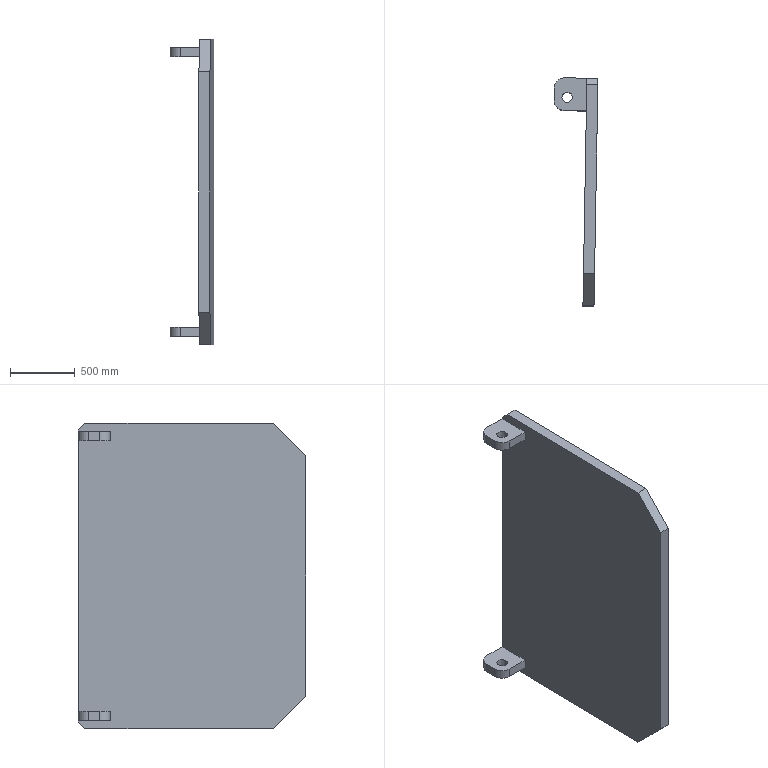Component | SolidWorks | BoxDoor-1 | 1 solid | 26 faces | box 337.93 x 1754.2 x 2350 mm | volume 351699217 mm3 | plane 18 | cylinder 8 | commonest cylinder face diameters 80 x4 160 x4
build123d program:
from build123d import *

# Parameters (mm, degrees)
BOSS_EXTRUDE1_DEPTH = 85
SKETCH2_W           = 70
SKETCH2_H           = 250
BOSS_EXTRUDE2_DEPTH = 250
CHAMFER1_SIZE       = 50
FILLET1_R           = 80
SKETCH3_R           = 40
CUT_EXTRUDE1_DEPTH  = 2460.543


with BuildPart() as part:
    # Sketch1 → Boss-Extrude1 (new body)
    with BuildSketch(Plane.XY):
        Polygon((-1175, -625), (-925, -875), (925, -875), (1175, -625), (1175, 875), (-1175, 875), align=None)
    extrude(amount=BOSS_EXTRUDE1_DEPTH)

    # Sketch2 → Boss-Extrude2 (add)
    with BuildSketch(Plane(origin=(0, 0, 0), x_dir=(-1, 0, 0), z_dir=(0, 0, -1))):
        with Locations((-1075, 750)):
            Rectangle(SKETCH2_W, SKETCH2_H)
        with Locations((1075, 750)):
            Rectangle(SKETCH2_W, SKETCH2_H)
    extrude(amount=BOSS_EXTRUDE2_DEPTH)

    # Chamfer1
    chamfer1_edges = [part.edges().sort_by_distance(p)[0] for p in [
        (-1175, 875, 42.5),
        (1175, 875, 42.5),
    ]]
    chamfer(chamfer1_edges, length=CHAMFER1_SIZE)

    # Fillet1
    fillet1_edges = [part.edges().sort_by_distance(p)[0] for p in [
        (1075, 625, -250),
        (1075, 875, -250),
        (-1075, 875, -250),
        (-1075, 625, -250),
    ]]
    fillet(fillet1_edges, radius=FILLET1_R)

    # Sketch3 → Cut-Extrude1 (cut, through all)
    with BuildSketch(Plane(origin=(1110, 0, 0), x_dir=(0, 0, -1), z_dir=(1, 0, 0))):
        with Locations(Location((150, 725, 0), (0, 0, 90))):
            Circle(SKETCH3_R)
    extrude(amount=-CUT_EXTRUDE1_DEPTH, mode=Mode.SUBTRACT)


solid = part.part

# Placed as in the assembly
solid = solid.moved(Location((1073.724, 2288.43, -62.386), (90, 88.999, -90)))
STEP:
#1=COLOUR_RGB('',0.7922,0.8196,0.9333);
#2=FILL_AREA_STYLE_COLOUR('',#1);
#3=FILL_AREA_STYLE('',(#2));
#4=SURFACE_STYLE_FILL_AREA(#3);
#5=SURFACE_SIDE_STYLE('',(#4));
#6=SURFACE_STYLE_USAGE(.BOTH.,#5);
#7=PRESENTATION_STYLE_ASSIGNMENT((#6));
#8=CARTESIAN_POINT('',(38.441,118.71,-43.401));
#9=VERTEX_POINT('',#8);
#10=CARTESIAN_POINT('',(35.292,118.765,-43.401));
#11=VERTEX_POINT('',#10);
#12=CARTESIAN_POINT('',(36.867,118.738,-43.401));
#13=DIRECTION('',(-0.,-0.,-1.));
#14=DIRECTION('',(0.01747,0.9998,-0.));
#15=AXIS2_PLACEMENT_3D('',#12,#13,#14);
#16=CIRCLE('',#15,1.575);
#17=EDGE_CURVE('',#9,#11,#16,.T.);
#18=ORIENTED_EDGE('',*,*,#17,.F.);
#19=CARTESIAN_POINT('',(38.441,118.71,-46.157));
#20=VERTEX_POINT('',#19);
#21=CARTESIAN_POINT('',(38.441,118.71,43.804));
#22=DIRECTION('',(-0.,0.,-1.));
#23=VECTOR('',#22,39.37);
#24=LINE('',#21,#23);
#25=EDGE_CURVE('',#9,#20,#24,.T.);
#26=ORIENTED_EDGE('',*,*,#25,.T.);
#27=CARTESIAN_POINT('',(35.292,118.765,-46.157));
#28=VERTEX_POINT('',#27);
#29=CARTESIAN_POINT('',(36.867,118.738,-46.157));
#30=DIRECTION('',(-0.,0.,-1.));
#31=DIRECTION('',(-0.9998,0.01747,0.));
#32=AXIS2_PLACEMENT_3D('',#29,#30,#31);
#33=CIRCLE('',#32,1.575);
#34=EDGE_CURVE('',#20,#28,#33,.T.);
#35=ORIENTED_EDGE('',*,*,#34,.T.);
#36=CARTESIAN_POINT('',(35.292,118.765,43.804));
#37=DIRECTION('',(-0.,0.,-1.));
#38=VECTOR('',#37,39.37);
#39=LINE('',#36,#38);
#40=EDGE_CURVE('',#11,#28,#39,.T.);
#41=ORIENTED_EDGE('',*,*,#40,.F.);
#42=EDGE_LOOP('',(#18,#26,#35,#41));
#43=FACE_OUTER_BOUND('',#42,.T.);
#44=CARTESIAN_POINT('',(36.867,118.738,43.804));
#45=DIRECTION('',(-0.,0.,-1.));
#46=DIRECTION('',(-0.9998,0.01747,0.));
#47=AXIS2_PLACEMENT_3D('',#44,#45,#46);
#48=CYLINDRICAL_SURFACE('',#47,1.575);
#49=ADVANCED_FACE('',(#43),#48,.F.);
#50=CARTESIAN_POINT('',(38.441,118.71,41.245));
#51=VERTEX_POINT('',#50);
#52=CARTESIAN_POINT('',(35.292,118.765,41.245));
#53=VERTEX_POINT('',#52);
#54=CARTESIAN_POINT('',(36.867,118.738,41.245));
#55=DIRECTION('',(-0.,-0.,-1.));
#56=DIRECTION('',(0.01747,0.9998,0.));
#57=AXIS2_PLACEMENT_3D('',#54,#55,#56);
#58=CIRCLE('',#57,1.575);
#59=EDGE_CURVE('',#51,#53,#58,.T.);
#60=ORIENTED_EDGE('',*,*,#59,.F.);
#61=CARTESIAN_POINT('',(38.441,118.71,38.489));
#62=VERTEX_POINT('',#61);
#63=CARTESIAN_POINT('',(38.441,118.71,43.804));
#64=DIRECTION('',(-0.,0.,-1.));
#65=VECTOR('',#64,39.37);
#66=LINE('',#63,#65);
#67=EDGE_CURVE('',#51,#62,#66,.T.);
#68=ORIENTED_EDGE('',*,*,#67,.T.);
#69=CARTESIAN_POINT('',(35.292,118.765,38.489));
#70=VERTEX_POINT('',#69);
#71=CARTESIAN_POINT('',(36.867,118.738,38.489));
#72=DIRECTION('',(-0.,-0.,1.));
#73=DIRECTION('',(-0.01747,-0.9998,-0.));
#74=AXIS2_PLACEMENT_3D('',#71,#72,#73);
#75=CIRCLE('',#74,1.575);
#76=EDGE_CURVE('',#70,#62,#75,.T.);
#77=ORIENTED_EDGE('',*,*,#76,.F.);
#78=CARTESIAN_POINT('',(35.292,118.765,43.804));
#79=DIRECTION('',(-0.,0.,-1.));
#80=VECTOR('',#79,39.37);
#81=LINE('',#78,#80);
#82=EDGE_CURVE('',#53,#70,#81,.T.);
#83=ORIENTED_EDGE('',*,*,#82,.F.);
#84=EDGE_LOOP('',(#60,#68,#77,#83));
#85=FACE_OUTER_BOUND('',#84,.T.);
#86=CARTESIAN_POINT('',(36.867,118.738,43.804));
#87=DIRECTION('',(-0.,0.,-1.));
#88=DIRECTION('',(-0.9998,0.01747,0.));
#89=AXIS2_PLACEMENT_3D('',#86,#87,#88);
#90=CYLINDRICAL_SURFACE('',#89,1.575);
#91=ADVANCED_FACE('',(#85),#90,.F.);
#92=CARTESIAN_POINT('',(42.84,122.571,43.804));
#93=VERTEX_POINT('',#92);
#94=CARTESIAN_POINT('',(41.843,65.493,43.804));
#95=VERTEX_POINT('',#94);
#96=CARTESIAN_POINT('',(42.874,124.539,43.804));
#97=DIRECTION('',(-0.01747,-0.9998,-0.));
#98=VECTOR('',#97,39.37);
#99=LINE('',#96,#98);
#100=EDGE_CURVE('',#93,#95,#99,.T.);
#101=ORIENTED_EDGE('',*,*,#100,.F.);
#102=CARTESIAN_POINT('',(42.874,124.539,41.835));
#103=VERTEX_POINT('',#102);
#104=CARTESIAN_POINT('',(42.84,122.571,43.804));
#105=DIRECTION('',(0.01235,0.707,-0.7071));
#106=VECTOR('',#105,39.37);
#107=LINE('',#104,#106);
#108=EDGE_CURVE('',#93,#103,#107,.T.);
#109=ORIENTED_EDGE('',*,*,#108,.T.);
#110=CARTESIAN_POINT('',(42.874,124.539,41.245));
#111=VERTEX_POINT('',#110);
#112=CARTESIAN_POINT('',(42.874,124.539,43.804));
#113=DIRECTION('',(0.,-0.,1.));
#114=VECTOR('',#113,39.37);
#115=LINE('',#112,#114);
#116=EDGE_CURVE('',#111,#103,#115,.T.);
#117=ORIENTED_EDGE('',*,*,#116,.F.);
#118=CARTESIAN_POINT('',(42.703,114.698,41.245));
#119=VERTEX_POINT('',#118);
#120=CARTESIAN_POINT('',(42.874,124.539,41.245));
#121=DIRECTION('',(0.01747,0.9998,-0.));
#122=VECTOR('',#121,39.37);
#123=LINE('',#120,#122);
#124=EDGE_CURVE('',#119,#111,#123,.T.);
#125=ORIENTED_EDGE('',*,*,#124,.F.);
#126=CARTESIAN_POINT('',(42.703,114.698,38.489));
#127=VERTEX_POINT('',#126);
#128=CARTESIAN_POINT('',(42.703,114.698,41.245));
#129=DIRECTION('',(0.,-0.,1.));
#130=VECTOR('',#129,39.37);
#131=LINE('',#128,#130);
#132=EDGE_CURVE('',#127,#119,#131,.T.);
#133=ORIENTED_EDGE('',*,*,#132,.F.);
#134=CARTESIAN_POINT('',(42.874,124.539,38.489));
#135=VERTEX_POINT('',#134);
#136=CARTESIAN_POINT('',(42.874,124.539,38.489));
#137=DIRECTION('',(-0.01747,-0.9998,-0.));
#138=VECTOR('',#137,39.37);
#139=LINE('',#136,#138);
#140=EDGE_CURVE('',#135,#127,#139,.T.);
#141=ORIENTED_EDGE('',*,*,#140,.F.);
#142=CARTESIAN_POINT('',(42.874,124.539,-43.401));
#143=VERTEX_POINT('',#142);
#144=CARTESIAN_POINT('',(42.874,124.539,43.804));
#145=DIRECTION('',(0.,-0.,1.));
#146=VECTOR('',#145,39.37);
#147=LINE('',#144,#146);
#148=EDGE_CURVE('',#143,#135,#147,.T.);
#149=ORIENTED_EDGE('',*,*,#148,.F.);
#150=CARTESIAN_POINT('',(42.703,114.698,-43.401));
#151=VERTEX_POINT('',#150);
#152=CARTESIAN_POINT('',(42.874,124.539,-43.401));
#153=DIRECTION('',(0.01747,0.9998,-0.));
#154=VECTOR('',#153,39.37);
#155=LINE('',#152,#154);
#156=EDGE_CURVE('',#151,#143,#155,.T.);
#157=ORIENTED_EDGE('',*,*,#156,.F.);
#158=CARTESIAN_POINT('',(42.703,114.698,-46.157));
#159=VERTEX_POINT('',#158);
#160=CARTESIAN_POINT('',(42.703,114.698,-46.157));
#161=DIRECTION('',(0.,-0.,1.));
#162=VECTOR('',#161,39.37);
#163=LINE('',#160,#162);
#164=EDGE_CURVE('',#159,#151,#163,.T.);
#165=ORIENTED_EDGE('',*,*,#164,.F.);
#166=CARTESIAN_POINT('',(42.874,124.539,-46.157));
#167=VERTEX_POINT('',#166);
#168=CARTESIAN_POINT('',(42.874,124.539,-46.157));
#169=DIRECTION('',(-0.01747,-0.9998,-0.));
#170=VECTOR('',#169,39.37);
#171=LINE('',#168,#170);
#172=EDGE_CURVE('',#167,#159,#171,.T.);
#173=ORIENTED_EDGE('',*,*,#172,.F.);
#174=CARTESIAN_POINT('',(42.874,124.539,-46.747));
#175=VERTEX_POINT('',#174);
#176=CARTESIAN_POINT('',(42.874,124.539,43.804));
#177=DIRECTION('',(0.,-0.,1.));
#178=VECTOR('',#177,39.37);
#179=LINE('',#176,#178);
#180=EDGE_CURVE('',#175,#167,#179,.T.);
#181=ORIENTED_EDGE('',*,*,#180,.F.);
#182=CARTESIAN_POINT('',(42.84,122.571,-48.716));
#183=VERTEX_POINT('',#182);
#184=CARTESIAN_POINT('',(42.874,124.539,-46.747));
#185=DIRECTION('',(-0.01235,-0.707,-0.7071));
#186=VECTOR('',#185,39.37);
#187=LINE('',#184,#186);
#188=EDGE_CURVE('',#175,#183,#187,.T.);
#189=ORIENTED_EDGE('',*,*,#188,.T.);
#190=CARTESIAN_POINT('',(41.843,65.493,-48.716));
#191=VERTEX_POINT('',#190);
#192=CARTESIAN_POINT('',(42.874,124.539,-48.716));
#193=DIRECTION('',(0.01747,0.9998,0.));
#194=VECTOR('',#193,39.37);
#195=LINE('',#192,#194);
#196=EDGE_CURVE('',#191,#183,#195,.T.);
#197=ORIENTED_EDGE('',*,*,#196,.F.);
#198=CARTESIAN_POINT('',(41.671,55.652,-38.873));
#199=VERTEX_POINT('',#198);
#200=CARTESIAN_POINT('',(41.671,55.652,-38.873));
#201=DIRECTION('',(0.01235,0.707,-0.7071));
#202=VECTOR('',#201,39.37);
#203=LINE('',#200,#202);
#204=EDGE_CURVE('',#199,#191,#203,.T.);
#205=ORIENTED_EDGE('',*,*,#204,.F.);
#206=CARTESIAN_POINT('',(41.671,55.652,33.961));
#207=VERTEX_POINT('',#206);
#208=CARTESIAN_POINT('',(41.671,55.652,33.961));
#209=DIRECTION('',(-0.,0.,-1.));
#210=VECTOR('',#209,39.37);
#211=LINE('',#208,#210);
#212=EDGE_CURVE('',#207,#199,#211,.T.);
#213=ORIENTED_EDGE('',*,*,#212,.F.);
#214=CARTESIAN_POINT('',(41.843,65.493,43.804));
#215=DIRECTION('',(-0.01235,-0.707,-0.7071));
#216=VECTOR('',#215,39.37);
#217=LINE('',#214,#216);
#218=EDGE_CURVE('',#95,#207,#217,.T.);
#219=ORIENTED_EDGE('',*,*,#218,.F.);
#220=EDGE_LOOP('',(#101,#109,#117,#125,#133,#141,#149,#157,#165,#173,#181,#189,#197,#205,#213,#219));
#221=FACE_OUTER_BOUND('',#220,.T.);
#222=CARTESIAN_POINT('',(42.273,90.096,-2.456));
#223=DIRECTION('',(0.9998,-0.01747,-0.));
#224=DIRECTION('',(-0.,0.,-1.));
#225=AXIS2_PLACEMENT_3D('',#222,#223,#224);
#226=PLANE('',#225);
#227=ADVANCED_FACE('',(#221),#226,.F.);
#228=CARTESIAN_POINT('',(46.186,122.513,43.804));
#229=VERTEX_POINT('',#228);
#230=CARTESIAN_POINT('',(45.189,65.435,43.804));
#231=VERTEX_POINT('',#230);
#232=CARTESIAN_POINT('',(46.22,124.481,43.804));
#233=DIRECTION('',(-0.01747,-0.9998,-0.));
#234=VECTOR('',#233,39.37);
#235=LINE('',#232,#234);
#236=EDGE_CURVE('',#229,#231,#235,.T.);
#237=ORIENTED_EDGE('',*,*,#236,.F.);
#238=CARTESIAN_POINT('',(46.186,122.513,43.804));
#239=DIRECTION('',(-0.9998,0.01747,0.));
#240=VECTOR('',#239,39.37);
#241=LINE('',#238,#240);
#242=EDGE_CURVE('',#229,#93,#241,.T.);
#243=ORIENTED_EDGE('',*,*,#242,.T.);
#244=ORIENTED_EDGE('',*,*,#100,.T.);
#245=CARTESIAN_POINT('',(45.189,65.435,43.804));
#246=DIRECTION('',(-0.9998,0.01747,0.));
#247=VECTOR('',#246,39.37);
#248=LINE('',#245,#247);
#249=EDGE_CURVE('',#231,#95,#248,.T.);
#250=ORIENTED_EDGE('',*,*,#249,.F.);
#251=EDGE_LOOP('',(#237,#243,#244,#250));
#252=FACE_OUTER_BOUND('',#251,.T.);
#253=CARTESIAN_POINT('',(46.22,124.481,43.804));
#254=DIRECTION('',(-0.,0.,-1.));
#255=DIRECTION('',(0.01747,0.9998,0.));
#256=AXIS2_PLACEMENT_3D('',#253,#254,#255);
#257=PLANE('',#256);
#258=ADVANCED_FACE('',(#252),#257,.F.);
#259=ORIENTED_EDGE('',*,*,#218,.T.);
#260=CARTESIAN_POINT('',(45.017,55.594,33.961));
#261=VERTEX_POINT('',#260);
#262=CARTESIAN_POINT('',(45.017,55.594,33.961));
#263=DIRECTION('',(-0.9998,0.01747,0.));
#264=VECTOR('',#263,39.37);
#265=LINE('',#262,#264);
#266=EDGE_CURVE('',#261,#207,#265,.T.);
#267=ORIENTED_EDGE('',*,*,#266,.F.);
#268=CARTESIAN_POINT('',(45.189,65.435,43.804));
#269=DIRECTION('',(-0.01235,-0.707,-0.7071));
#270=VECTOR('',#269,39.37);
#271=LINE('',#268,#270);
#272=EDGE_CURVE('',#231,#261,#271,.T.);
#273=ORIENTED_EDGE('',*,*,#272,.F.);
#274=ORIENTED_EDGE('',*,*,#249,.T.);
#275=EDGE_LOOP('',(#259,#267,#273,#274));
#276=FACE_OUTER_BOUND('',#275,.T.);
#277=CARTESIAN_POINT('',(45.189,65.435,43.804));
#278=DIRECTION('',(0.01235,0.707,-0.7071));
#279=DIRECTION('',(0.01235,0.707,0.7071));
#280=AXIS2_PLACEMENT_3D('',#277,#278,#279);
#281=PLANE('',#280);
#282=ADVANCED_FACE('',(#276),#281,.F.);
#283=ORIENTED_EDGE('',*,*,#212,.T.);
#284=CARTESIAN_POINT('',(45.017,55.594,-38.873));
#285=VERTEX_POINT('',#284);
#286=CARTESIAN_POINT('',(45.017,55.594,-38.873));
#287=DIRECTION('',(-0.9998,0.01747,0.));
#288=VECTOR('',#287,39.37);
#289=LINE('',#286,#288);
#290=EDGE_CURVE('',#285,#199,#289,.T.);
#291=ORIENTED_EDGE('',*,*,#290,.F.);
#292=CARTESIAN_POINT('',(45.017,55.594,33.961));
#293=DIRECTION('',(-0.,0.,-1.));
#294=VECTOR('',#293,39.37);
#295=LINE('',#292,#294);
#296=EDGE_CURVE('',#261,#285,#295,.T.);
#297=ORIENTED_EDGE('',*,*,#296,.F.);
#298=ORIENTED_EDGE('',*,*,#266,.T.);
#299=EDGE_LOOP('',(#283,#291,#297,#298));
#300=FACE_OUTER_BOUND('',#299,.T.);
#301=CARTESIAN_POINT('',(45.017,55.594,33.961));
#302=DIRECTION('',(0.01747,0.9998,0.));
#303=DIRECTION('',(0.9998,-0.01747,-0.));
#304=AXIS2_PLACEMENT_3D('',#301,#302,#303);
#305=PLANE('',#304);
#306=ADVANCED_FACE('',(#300),#305,.F.);
#307=ORIENTED_EDGE('',*,*,#204,.T.);
#308=CARTESIAN_POINT('',(45.189,65.435,-48.716));
#309=VERTEX_POINT('',#308);
#310=CARTESIAN_POINT('',(45.189,65.435,-48.716));
#311=DIRECTION('',(-0.9998,0.01747,0.));
#312=VECTOR('',#311,39.37);
#313=LINE('',#310,#312);
#314=EDGE_CURVE('',#309,#191,#313,.T.);
#315=ORIENTED_EDGE('',*,*,#314,.F.);
#316=CARTESIAN_POINT('',(45.017,55.594,-38.873));
#317=DIRECTION('',(0.01235,0.707,-0.7071));
#318=VECTOR('',#317,39.37);
#319=LINE('',#316,#318);
#320=EDGE_CURVE('',#285,#309,#319,.T.);
#321=ORIENTED_EDGE('',*,*,#320,.F.);
#322=ORIENTED_EDGE('',*,*,#290,.T.);
#323=EDGE_LOOP('',(#307,#315,#321,#322));
#324=FACE_OUTER_BOUND('',#323,.T.);
#325=CARTESIAN_POINT('',(45.017,55.594,-38.873));
#326=DIRECTION('',(0.01235,0.707,0.7071));
#327=DIRECTION('',(-0.01235,-0.707,0.7071));
#328=AXIS2_PLACEMENT_3D('',#325,#326,#327);
#329=PLANE('',#328);
#330=ADVANCED_FACE('',(#324),#329,.F.);
#331=ORIENTED_EDGE('',*,*,#196,.T.);
#332=CARTESIAN_POINT('',(46.186,122.513,-48.716));
#333=VERTEX_POINT('',#332);
#334=CARTESIAN_POINT('',(46.186,122.513,-48.716));
#335=DIRECTION('',(0.9998,-0.01747,-0.));
#336=VECTOR('',#335,39.37);
#337=LINE('',#334,#336);
#338=EDGE_CURVE('',#183,#333,#337,.T.);
#339=ORIENTED_EDGE('',*,*,#338,.T.);
#340=CARTESIAN_POINT('',(46.22,124.481,-48.716));
#341=DIRECTION('',(0.01747,0.9998,0.));
#342=VECTOR('',#341,39.37);
#343=LINE('',#340,#342);
#344=EDGE_CURVE('',#309,#333,#343,.T.);
#345=ORIENTED_EDGE('',*,*,#344,.F.);
#346=ORIENTED_EDGE('',*,*,#314,.T.);
#347=EDGE_LOOP('',(#331,#339,#345,#346));
#348=FACE_OUTER_BOUND('',#347,.T.);
#349=CARTESIAN_POINT('',(46.22,124.481,-48.716));
#350=DIRECTION('',(0.,-0.,1.));
#351=DIRECTION('',(-0.01747,-0.9998,-0.));
#352=AXIS2_PLACEMENT_3D('',#349,#350,#351);
#353=PLANE('',#352);
#354=ADVANCED_FACE('',(#348),#353,.F.);
#355=CARTESIAN_POINT('',(36.183,124.656,38.489));
#356=VERTEX_POINT('',#355);
#357=CARTESIAN_POINT('',(33.033,124.711,38.489));
#358=DIRECTION('',(0.9998,-0.01747,-0.));
#359=VECTOR('',#358,39.37);
#360=LINE('',#357,#359);
#361=EDGE_CURVE('',#356,#135,#360,.T.);
#362=ORIENTED_EDGE('',*,*,#361,.F.);
#363=CARTESIAN_POINT('',(36.183,124.656,41.245));
#364=VERTEX_POINT('',#363);
#365=CARTESIAN_POINT('',(36.183,124.656,41.245));
#366=DIRECTION('',(0.,-0.,1.));
#367=VECTOR('',#366,39.37);
#368=LINE('',#365,#367);
#369=EDGE_CURVE('',#356,#364,#368,.T.);
#370=ORIENTED_EDGE('',*,*,#369,.T.);
#371=CARTESIAN_POINT('',(33.033,124.711,41.245));
#372=DIRECTION('',(0.9998,-0.01747,-0.));
#373=VECTOR('',#372,39.37);
#374=LINE('',#371,#373);
#375=EDGE_CURVE('',#364,#111,#374,.T.);
#376=ORIENTED_EDGE('',*,*,#375,.T.);
#377=ORIENTED_EDGE('',*,*,#116,.T.);
#378=CARTESIAN_POINT('',(46.22,124.481,41.835));
#379=VERTEX_POINT('',#378);
#380=CARTESIAN_POINT('',(46.22,124.481,41.835));
#381=DIRECTION('',(0.9998,-0.01747,-0.));
#382=VECTOR('',#381,39.37);
#383=LINE('',#380,#382);
#384=EDGE_CURVE('',#103,#379,#383,.T.);
#385=ORIENTED_EDGE('',*,*,#384,.T.);
#386=CARTESIAN_POINT('',(46.22,124.481,-46.747));
#387=VERTEX_POINT('',#386);
#388=CARTESIAN_POINT('',(46.22,124.481,43.804));
#389=DIRECTION('',(0.,-0.,1.));
#390=VECTOR('',#389,39.37);
#391=LINE('',#388,#390);
#392=EDGE_CURVE('',#387,#379,#391,.T.);
#393=ORIENTED_EDGE('',*,*,#392,.F.);
#394=CARTESIAN_POINT('',(46.22,124.481,-46.747));
#395=DIRECTION('',(-0.9998,0.01747,0.));
#396=VECTOR('',#395,39.37);
#397=LINE('',#394,#396);
#398=EDGE_CURVE('',#387,#175,#397,.T.);
#399=ORIENTED_EDGE('',*,*,#398,.T.);
#400=ORIENTED_EDGE('',*,*,#180,.T.);
#401=CARTESIAN_POINT('',(36.183,124.656,-46.157));
#402=VERTEX_POINT('',#401);
#403=CARTESIAN_POINT('',(33.033,124.711,-46.157));
#404=DIRECTION('',(0.9998,-0.01747,-0.));
#405=VECTOR('',#404,39.37);
#406=LINE('',#403,#405);
#407=EDGE_CURVE('',#402,#167,#406,.T.);
#408=ORIENTED_EDGE('',*,*,#407,.F.);
#409=CARTESIAN_POINT('',(36.183,124.656,-43.401));
#410=VERTEX_POINT('',#409);
#411=CARTESIAN_POINT('',(36.183,124.656,-43.401));
#412=DIRECTION('',(0.,-0.,1.));
#413=VECTOR('',#412,39.37);
#414=LINE('',#411,#413);
#415=EDGE_CURVE('',#402,#410,#414,.T.);
#416=ORIENTED_EDGE('',*,*,#415,.T.);
#417=CARTESIAN_POINT('',(33.033,124.711,-43.401));
#418=DIRECTION('',(0.9998,-0.01747,-0.));
#419=VECTOR('',#418,39.37);
#420=LINE('',#417,#419);
#421=EDGE_CURVE('',#410,#143,#420,.T.);
#422=ORIENTED_EDGE('',*,*,#421,.T.);
#423=ORIENTED_EDGE('',*,*,#148,.T.);
#424=EDGE_LOOP('',(#362,#370,#376,#377,#385,#393,#399,#400,#408,#416,#422,#423));
#425=FACE_OUTER_BOUND('',#424,.T.);
#426=CARTESIAN_POINT('',(46.22,124.481,43.804));
#427=DIRECTION('',(-0.01747,-0.9998,-0.));
#428=DIRECTION('',(-0.9998,0.01747,0.));
#429=AXIS2_PLACEMENT_3D('',#426,#427,#428);
#430=PLANE('',#429);
#431=ADVANCED_FACE('',(#425),#430,.F.);
#432=ORIENTED_EDGE('',*,*,#392,.T.);
#433=CARTESIAN_POINT('',(46.306,129.401,36.914));
#434=DIRECTION('',(-0.01235,-0.707,0.7071));
#435=VECTOR('',#434,39.37);
#436=LINE('',#433,#435);
#437=EDGE_CURVE('',#379,#229,#436,.T.);
#438=ORIENTED_EDGE('',*,*,#437,.T.);
#439=ORIENTED_EDGE('',*,*,#236,.T.);
#440=ORIENTED_EDGE('',*,*,#272,.T.);
#441=ORIENTED_EDGE('',*,*,#296,.T.);
#442=ORIENTED_EDGE('',*,*,#320,.T.);
#443=ORIENTED_EDGE('',*,*,#344,.T.);
#444=CARTESIAN_POINT('',(46.306,129.401,-41.826));
#445=DIRECTION('',(0.01235,0.707,0.7071));
#446=VECTOR('',#445,39.37);
#447=LINE('',#444,#446);
#448=EDGE_CURVE('',#333,#387,#447,.T.);
#449=ORIENTED_EDGE('',*,*,#448,.T.);
#450=EDGE_LOOP('',(#432,#438,#439,#440,#441,#442,#443,#449));
#451=FACE_OUTER_BOUND('',#450,.T.);
#452=CARTESIAN_POINT('',(45.619,90.037,-2.456));
#453=DIRECTION('',(0.9998,-0.01747,-0.));
#454=DIRECTION('',(-0.,0.,-1.));
#455=AXIS2_PLACEMENT_3D('',#452,#453,#454);
#456=PLANE('',#455);
#457=ADVANCED_FACE('',(#451),#456,.T.);
#458=CARTESIAN_POINT('',(36.867,118.738,-46.157));
#459=DIRECTION('',(-0.,0.,-1.));
#460=DIRECTION('',(-0.9998,0.01747,0.));
#461=AXIS2_PLACEMENT_3D('',#458,#459,#460);
#462=CIRCLE('',#461,1.575);
#463=EDGE_CURVE('',#28,#20,#462,.T.);
#464=ORIENTED_EDGE('',*,*,#463,.F.);
#465=ORIENTED_EDGE('',*,*,#34,.F.);
#466=EDGE_LOOP('',(#464,#465));
#467=FACE_BOUND('',#466,.T.);
#468=CARTESIAN_POINT('',(36.011,114.815,-46.157));
#469=VERTEX_POINT('',#468);
#470=CARTESIAN_POINT('',(32.861,114.87,-46.157));
#471=DIRECTION('',(0.9998,-0.01747,-0.));
#472=VECTOR('',#471,39.37);
#473=LINE('',#470,#472);
#474=EDGE_CURVE('',#469,#159,#473,.T.);
#475=ORIENTED_EDGE('',*,*,#474,.F.);
#476=CARTESIAN_POINT('',(32.917,118.019,-46.157));
#477=VERTEX_POINT('',#476);
#478=CARTESIAN_POINT('',(36.066,117.964,-46.157));
#479=DIRECTION('',(-0.,0.,-1.));
#480=DIRECTION('',(-0.01747,-0.9998,0.));
#481=AXIS2_PLACEMENT_3D('',#478,#479,#480);
#482=CIRCLE('',#481,3.15);
#483=EDGE_CURVE('',#469,#477,#482,.T.);
#484=ORIENTED_EDGE('',*,*,#483,.T.);
#485=CARTESIAN_POINT('',(32.978,121.562,-46.157));
#486=VERTEX_POINT('',#485);
#487=CARTESIAN_POINT('',(33.033,124.711,-46.157));
#488=DIRECTION('',(-0.01747,-0.9998,-0.));
#489=VECTOR('',#488,39.37);
#490=LINE('',#487,#489);
#491=EDGE_CURVE('',#486,#477,#490,.T.);
#492=ORIENTED_EDGE('',*,*,#491,.F.);
#493=CARTESIAN_POINT('',(36.128,121.507,-46.157));
#494=DIRECTION('',(-0.,0.,-1.));
#495=DIRECTION('',(-0.01747,-0.9998,0.));
#496=AXIS2_PLACEMENT_3D('',#493,#494,#495);
#497=CIRCLE('',#496,3.15);
#498=EDGE_CURVE('',#486,#402,#497,.T.);
#499=ORIENTED_EDGE('',*,*,#498,.T.);
#500=ORIENTED_EDGE('',*,*,#407,.T.);
#501=ORIENTED_EDGE('',*,*,#172,.T.);
#502=EDGE_LOOP('',(#475,#484,#492,#499,#500,#501));
#503=FACE_OUTER_BOUND('',#502,.T.);
#504=CARTESIAN_POINT('',(33.033,124.711,-46.157));
#505=DIRECTION('',(0.,-0.,1.));
#506=DIRECTION('',(-0.01747,-0.9998,-0.));
#507=AXIS2_PLACEMENT_3D('',#504,#505,#506);
#508=PLANE('',#507);
#509=ADVANCED_FACE('',(#467,#503),#508,.F.);
#510=CARTESIAN_POINT('',(36.011,114.815,-43.401));
#511=VERTEX_POINT('',#510);
#512=CARTESIAN_POINT('',(32.861,114.87,-43.401));
#513=DIRECTION('',(0.9998,-0.01747,-0.));
#514=VECTOR('',#513,39.37);
#515=LINE('',#512,#514);
#516=EDGE_CURVE('',#511,#151,#515,.T.);
#517=ORIENTED_EDGE('',*,*,#516,.F.);
#518=CARTESIAN_POINT('',(36.011,114.815,-46.157));
#519=DIRECTION('',(-0.,0.,-1.));
#520=VECTOR('',#519,39.37);
#521=LINE('',#518,#520);
#522=EDGE_CURVE('',#511,#469,#521,.T.);
#523=ORIENTED_EDGE('',*,*,#522,.T.);
#524=ORIENTED_EDGE('',*,*,#474,.T.);
#525=ORIENTED_EDGE('',*,*,#164,.T.);
#526=EDGE_LOOP('',(#517,#523,#524,#525));
#527=FACE_OUTER_BOUND('',#526,.T.);
#528=CARTESIAN_POINT('',(32.861,114.87,-46.157));
#529=DIRECTION('',(0.01747,0.9998,0.));
#530=DIRECTION('',(0.9998,-0.01747,-0.));
#531=AXIS2_PLACEMENT_3D('',#528,#529,#530);
#532=PLANE('',#531);
#533=ADVANCED_FACE('',(#527),#532,.F.);
#534=CARTESIAN_POINT('',(36.867,118.738,-43.401));
#535=DIRECTION('',(-0.,-0.,-1.));
#536=DIRECTION('',(0.01747,0.9998,-0.));
#537=AXIS2_PLACEMENT_3D('',#534,#535,#536);
#538=CIRCLE('',#537,1.575);
#539=EDGE_CURVE('',#11,#9,#538,.T.);
#540=ORIENTED_EDGE('',*,*,#539,.T.);
#541=ORIENTED_EDGE('',*,*,#17,.T.);
#542=EDGE_LOOP('',(#540,#541));
#543=FACE_BOUND('',#542,.T.);
#544=CARTESIAN_POINT('',(32.917,118.019,-43.401));
#545=VERTEX_POINT('',#544);
#546=CARTESIAN_POINT('',(32.978,121.562,-43.401));
#547=VERTEX_POINT('',#546);
#548=CARTESIAN_POINT('',(33.033,124.711,-43.401));
#549=DIRECTION('',(0.01747,0.9998,-0.));
#550=VECTOR('',#549,39.37);
#551=LINE('',#548,#550);
#552=EDGE_CURVE('',#545,#547,#551,.T.);
#553=ORIENTED_EDGE('',*,*,#552,.F.);
#554=CARTESIAN_POINT('',(36.066,117.964,-43.401));
#555=DIRECTION('',(0.,0.,1.));
#556=DIRECTION('',(0.01747,0.9998,-0.));
#557=AXIS2_PLACEMENT_3D('',#554,#555,#556);
#558=CIRCLE('',#557,3.15);
#559=EDGE_CURVE('',#545,#511,#558,.T.);
#560=ORIENTED_EDGE('',*,*,#559,.T.);
#561=ORIENTED_EDGE('',*,*,#516,.T.);
#562=ORIENTED_EDGE('',*,*,#156,.T.);
#563=ORIENTED_EDGE('',*,*,#421,.F.);
#564=CARTESIAN_POINT('',(36.128,121.507,-43.401));
#565=DIRECTION('',(0.,0.,1.));
#566=DIRECTION('',(0.01747,0.9998,-0.));
#567=AXIS2_PLACEMENT_3D('',#564,#565,#566);
#568=CIRCLE('',#567,3.15);
#569=EDGE_CURVE('',#410,#547,#568,.T.);
#570=ORIENTED_EDGE('',*,*,#569,.T.);
#571=EDGE_LOOP('',(#553,#560,#561,#562,#563,#570));
#572=FACE_OUTER_BOUND('',#571,.T.);
#573=CARTESIAN_POINT('',(33.033,124.711,-43.401));
#574=DIRECTION('',(-0.,-0.,-1.));
#575=DIRECTION('',(0.01747,0.9998,-0.));
#576=AXIS2_PLACEMENT_3D('',#573,#574,#575);
#577=PLANE('',#576);
#578=ADVANCED_FACE('',(#543,#572),#577,.F.);
#579=ORIENTED_EDGE('',*,*,#491,.T.);
#580=CARTESIAN_POINT('',(32.917,118.019,-43.401));
#581=DIRECTION('',(0.,-0.,1.));
#582=VECTOR('',#581,39.37);
#583=LINE('',#580,#582);
#584=EDGE_CURVE('',#477,#545,#583,.T.);
#585=ORIENTED_EDGE('',*,*,#584,.T.);
#586=ORIENTED_EDGE('',*,*,#552,.T.);
#587=CARTESIAN_POINT('',(32.978,121.562,-46.157));
#588=DIRECTION('',(-0.,0.,-1.));
#589=VECTOR('',#588,39.37);
#590=LINE('',#587,#589);
#591=EDGE_CURVE('',#547,#486,#590,.T.);
#592=ORIENTED_EDGE('',*,*,#591,.T.);
#593=EDGE_LOOP('',(#579,#585,#586,#592));
#594=FACE_OUTER_BOUND('',#593,.T.);
#595=CARTESIAN_POINT('',(32.432,90.268,-2.456));
#596=DIRECTION('',(-0.9998,0.01747,0.));
#597=DIRECTION('',(0.,-0.,1.));
#598=AXIS2_PLACEMENT_3D('',#595,#596,#597);
#599=PLANE('',#598);
#600=ADVANCED_FACE('',(#594),#599,.T.);
#601=ORIENTED_EDGE('',*,*,#76,.T.);
#602=CARTESIAN_POINT('',(36.867,118.738,38.489));
#603=DIRECTION('',(-0.,-0.,1.));
#604=DIRECTION('',(-0.01747,-0.9998,-0.));
#605=AXIS2_PLACEMENT_3D('',#602,#603,#604);
#606=CIRCLE('',#605,1.575);
#607=EDGE_CURVE('',#62,#70,#606,.T.);
#608=ORIENTED_EDGE('',*,*,#607,.T.);
#609=EDGE_LOOP('',(#601,#608));
#610=FACE_BOUND('',#609,.T.);
#611=CARTESIAN_POINT('',(36.011,114.815,38.489));
#612=VERTEX_POINT('',#611);
#613=CARTESIAN_POINT('',(32.861,114.87,38.489));
#614=DIRECTION('',(0.9998,-0.01747,-0.));
#615=VECTOR('',#614,39.37);
#616=LINE('',#613,#615);
#617=EDGE_CURVE('',#612,#127,#616,.T.);
#618=ORIENTED_EDGE('',*,*,#617,.F.);
#619=CARTESIAN_POINT('',(32.917,118.019,38.489));
#620=VERTEX_POINT('',#619);
#621=CARTESIAN_POINT('',(36.066,117.964,38.489));
#622=DIRECTION('',(0.,0.,-1.));
#623=DIRECTION('',(-0.01747,-0.9998,-0.));
#624=AXIS2_PLACEMENT_3D('',#621,#622,#623);
#625=CIRCLE('',#624,3.15);
#626=EDGE_CURVE('',#612,#620,#625,.T.);
#627=ORIENTED_EDGE('',*,*,#626,.T.);
#628=CARTESIAN_POINT('',(32.978,121.562,38.489));
#629=VERTEX_POINT('',#628);
#630=CARTESIAN_POINT('',(33.033,124.711,38.489));
#631=DIRECTION('',(-0.01747,-0.9998,-0.));
#632=VECTOR('',#631,39.37);
#633=LINE('',#630,#632);
#634=EDGE_CURVE('',#629,#620,#633,.T.);
#635=ORIENTED_EDGE('',*,*,#634,.F.);
#636=CARTESIAN_POINT('',(36.128,121.507,38.489));
#637=DIRECTION('',(0.,0.,-1.));
#638=DIRECTION('',(-0.01747,-0.9998,-0.));
#639=AXIS2_PLACEMENT_3D('',#636,#637,#638);
#640=CIRCLE('',#639,3.15);
#641=EDGE_CURVE('',#629,#356,#640,.T.);
#642=ORIENTED_EDGE('',*,*,#641,.T.);
#643=ORIENTED_EDGE('',*,*,#361,.T.);
#644=ORIENTED_EDGE('',*,*,#140,.T.);
#645=EDGE_LOOP('',(#618,#627,#635,#642,#643,#644));
#646=FACE_OUTER_BOUND('',#645,.T.);
#647=CARTESIAN_POINT('',(33.033,124.711,38.489));
#648=DIRECTION('',(-0.,-0.,1.));
#649=DIRECTION('',(-0.01747,-0.9998,-0.));
#650=AXIS2_PLACEMENT_3D('',#647,#648,#649);
#651=PLANE('',#650);
#652=ADVANCED_FACE('',(#610,#646),#651,.F.);
#653=CARTESIAN_POINT('',(36.011,114.815,41.245));
#654=VERTEX_POINT('',#653);
#655=CARTESIAN_POINT('',(32.861,114.87,41.245));
#656=DIRECTION('',(0.9998,-0.01747,-0.));
#657=VECTOR('',#656,39.37);
#658=LINE('',#655,#657);
#659=EDGE_CURVE('',#654,#119,#658,.T.);
#660=ORIENTED_EDGE('',*,*,#659,.F.);
#661=CARTESIAN_POINT('',(36.011,114.815,38.489));
#662=DIRECTION('',(-0.,0.,-1.));
#663=VECTOR('',#662,39.37);
#664=LINE('',#661,#663);
#665=EDGE_CURVE('',#654,#612,#664,.T.);
#666=ORIENTED_EDGE('',*,*,#665,.T.);
#667=ORIENTED_EDGE('',*,*,#617,.T.);
#668=ORIENTED_EDGE('',*,*,#132,.T.);
#669=EDGE_LOOP('',(#660,#666,#667,#668));
#670=FACE_OUTER_BOUND('',#669,.T.);
#671=CARTESIAN_POINT('',(32.861,114.87,41.245));
#672=DIRECTION('',(0.01747,0.9998,0.));
#673=DIRECTION('',(0.9998,-0.01747,-0.));
#674=AXIS2_PLACEMENT_3D('',#671,#672,#673);
#675=PLANE('',#674);
#676=ADVANCED_FACE('',(#670),#675,.F.);
#677=CARTESIAN_POINT('',(36.867,118.738,41.245));
#678=DIRECTION('',(-0.,-0.,-1.));
#679=DIRECTION('',(0.01747,0.9998,0.));
#680=AXIS2_PLACEMENT_3D('',#677,#678,#679);
#681=CIRCLE('',#680,1.575);
#682=EDGE_CURVE('',#53,#51,#681,.T.);
#683=ORIENTED_EDGE('',*,*,#682,.T.);
#684=ORIENTED_EDGE('',*,*,#59,.T.);
#685=EDGE_LOOP('',(#683,#684));
#686=FACE_BOUND('',#685,.T.);
#687=CARTESIAN_POINT('',(32.917,118.019,41.245));
#688=VERTEX_POINT('',#687);
#689=CARTESIAN_POINT('',(32.978,121.562,41.245));
#690=VERTEX_POINT('',#689);
#691=CARTESIAN_POINT('',(33.033,124.711,41.245));
#692=DIRECTION('',(0.01747,0.9998,-0.));
#693=VECTOR('',#692,39.37);
#694=LINE('',#691,#693);
#695=EDGE_CURVE('',#688,#690,#694,.T.);
#696=ORIENTED_EDGE('',*,*,#695,.F.);
#697=CARTESIAN_POINT('',(36.066,117.964,41.245));
#698=DIRECTION('',(0.,0.,1.));
#699=DIRECTION('',(0.01747,0.9998,-0.));
#700=AXIS2_PLACEMENT_3D('',#697,#698,#699);
#701=CIRCLE('',#700,3.15);
#702=EDGE_CURVE('',#688,#654,#701,.T.);
#703=ORIENTED_EDGE('',*,*,#702,.T.);
#704=ORIENTED_EDGE('',*,*,#659,.T.);
#705=ORIENTED_EDGE('',*,*,#124,.T.);
#706=ORIENTED_EDGE('',*,*,#375,.F.);
#707=CARTESIAN_POINT('',(36.128,121.507,41.245));
#708=DIRECTION('',(0.,0.,1.));
#709=DIRECTION('',(0.01747,0.9998,-0.));
#710=AXIS2_PLACEMENT_3D('',#707,#708,#709);
#711=CIRCLE('',#710,3.15);
#712=EDGE_CURVE('',#364,#690,#711,.T.);
#713=ORIENTED_EDGE('',*,*,#712,.T.);
#714=EDGE_LOOP('',(#696,#703,#704,#705,#706,#713));
#715=FACE_OUTER_BOUND('',#714,.T.);
#716=CARTESIAN_POINT('',(33.033,124.711,41.245));
#717=DIRECTION('',(-0.,-0.,-1.));
#718=DIRECTION('',(0.01747,0.9998,-0.));
#719=AXIS2_PLACEMENT_3D('',#716,#717,#718);
#720=PLANE('',#719);
#721=ADVANCED_FACE('',(#686,#715),#720,.F.);
#722=ORIENTED_EDGE('',*,*,#634,.T.);
#723=CARTESIAN_POINT('',(32.917,118.019,41.245));
#724=DIRECTION('',(0.,-0.,1.));
#725=VECTOR('',#724,39.37);
#726=LINE('',#723,#725);
#727=EDGE_CURVE('',#620,#688,#726,.T.);
#728=ORIENTED_EDGE('',*,*,#727,.T.);
#729=ORIENTED_EDGE('',*,*,#695,.T.);
#730=CARTESIAN_POINT('',(32.978,121.562,38.489));
#731=DIRECTION('',(-0.,0.,-1.));
#732=VECTOR('',#731,39.37);
#733=LINE('',#730,#732);
#734=EDGE_CURVE('',#690,#629,#733,.T.);
#735=ORIENTED_EDGE('',*,*,#734,.T.);
#736=EDGE_LOOP('',(#722,#728,#729,#735));
#737=FACE_OUTER_BOUND('',#736,.T.);
#738=CARTESIAN_POINT('',(32.432,90.268,-2.456));
#739=DIRECTION('',(-0.9998,0.01747,0.));
#740=DIRECTION('',(0.,-0.,1.));
#741=AXIS2_PLACEMENT_3D('',#738,#739,#740);
#742=PLANE('',#741);
#743=ADVANCED_FACE('',(#737),#742,.T.);
#744=ORIENTED_EDGE('',*,*,#437,.F.);
#745=ORIENTED_EDGE('',*,*,#384,.F.);
#746=ORIENTED_EDGE('',*,*,#108,.F.);
#747=ORIENTED_EDGE('',*,*,#242,.F.);
#748=EDGE_LOOP('',(#744,#745,#746,#747));
#749=FACE_OUTER_BOUND('',#748,.T.);
#750=CARTESIAN_POINT('',(46.186,122.513,43.804));
#751=DIRECTION('',(-0.01235,-0.707,-0.7071));
#752=DIRECTION('',(-0.9998,0.01747,0.));
#753=AXIS2_PLACEMENT_3D('',#750,#751,#752);
#754=PLANE('',#753);
#755=ADVANCED_FACE('',(#749),#754,.F.);
#756=ORIENTED_EDGE('',*,*,#448,.F.);
#757=ORIENTED_EDGE('',*,*,#338,.F.);
#758=ORIENTED_EDGE('',*,*,#188,.F.);
#759=ORIENTED_EDGE('',*,*,#398,.F.);
#760=EDGE_LOOP('',(#756,#757,#758,#759));
#761=FACE_OUTER_BOUND('',#760,.T.);
#762=CARTESIAN_POINT('',(46.22,124.481,-46.747));
#763=DIRECTION('',(-0.01235,-0.707,0.7071));
#764=DIRECTION('',(-0.9998,0.01747,0.));
#765=AXIS2_PLACEMENT_3D('',#762,#763,#764);
#766=PLANE('',#765);
#767=ADVANCED_FACE('',(#761),#766,.F.);
#768=ORIENTED_EDGE('',*,*,#626,.F.);
#769=ORIENTED_EDGE('',*,*,#665,.F.);
#770=ORIENTED_EDGE('',*,*,#702,.F.);
#771=ORIENTED_EDGE('',*,*,#727,.F.);
#772=EDGE_LOOP('',(#768,#769,#770,#771));
#773=FACE_OUTER_BOUND('',#772,.T.);
#774=CARTESIAN_POINT('',(36.066,117.964,-2.456));
#775=DIRECTION('',(-0.,0.,-1.));
#776=DIRECTION('',(-0.9998,0.01747,0.));
#777=AXIS2_PLACEMENT_3D('',#774,#775,#776);
#778=CYLINDRICAL_SURFACE('',#777,3.15);
#779=ADVANCED_FACE('',(#773),#778,.T.);
#780=ORIENTED_EDGE('',*,*,#712,.F.);
#781=ORIENTED_EDGE('',*,*,#369,.F.);
#782=ORIENTED_EDGE('',*,*,#641,.F.);
#783=ORIENTED_EDGE('',*,*,#734,.F.);
#784=EDGE_LOOP('',(#780,#781,#782,#783));
#785=FACE_OUTER_BOUND('',#784,.T.);
#786=CARTESIAN_POINT('',(36.128,121.507,-2.456));
#787=DIRECTION('',(0.,-0.,1.));
#788=DIRECTION('',(0.9998,-0.01747,0.));
#789=AXIS2_PLACEMENT_3D('',#786,#787,#788);
#790=CYLINDRICAL_SURFACE('',#789,3.15);
#791=ADVANCED_FACE('',(#785),#790,.T.);
#792=ORIENTED_EDGE('',*,*,#483,.F.);
#793=ORIENTED_EDGE('',*,*,#522,.F.);
#794=ORIENTED_EDGE('',*,*,#559,.F.);
#795=ORIENTED_EDGE('',*,*,#584,.F.);
#796=EDGE_LOOP('',(#792,#793,#794,#795));
#797=FACE_OUTER_BOUND('',#796,.T.);
#798=CARTESIAN_POINT('',(36.066,117.964,-2.456));
#799=DIRECTION('',(-0.,0.,-1.));
#800=DIRECTION('',(-0.9998,0.01747,0.));
#801=AXIS2_PLACEMENT_3D('',#798,#799,#800);
#802=CYLINDRICAL_SURFACE('',#801,3.15);
#803=ADVANCED_FACE('',(#797),#802,.T.);
#804=ORIENTED_EDGE('',*,*,#569,.F.);
#805=ORIENTED_EDGE('',*,*,#415,.F.);
#806=ORIENTED_EDGE('',*,*,#498,.F.);
#807=ORIENTED_EDGE('',*,*,#591,.F.);
#808=EDGE_LOOP('',(#804,#805,#806,#807));
#809=FACE_OUTER_BOUND('',#808,.T.);
#810=CARTESIAN_POINT('',(36.128,121.507,-2.456));
#811=DIRECTION('',(0.,-0.,1.));
#812=DIRECTION('',(0.9998,-0.01747,0.));
#813=AXIS2_PLACEMENT_3D('',#810,#811,#812);
#814=CYLINDRICAL_SURFACE('',#813,3.15);
#815=ADVANCED_FACE('',(#809),#814,.T.);
#816=ORIENTED_EDGE('',*,*,#67,.F.);
#817=ORIENTED_EDGE('',*,*,#682,.F.);
#818=ORIENTED_EDGE('',*,*,#82,.T.);
#819=ORIENTED_EDGE('',*,*,#607,.F.);
#820=EDGE_LOOP('',(#816,#817,#818,#819));
#821=FACE_OUTER_BOUND('',#820,.T.);
#822=CARTESIAN_POINT('',(36.867,118.738,43.804));
#823=DIRECTION('',(-0.,0.,-1.));
#824=DIRECTION('',(-0.9998,0.01747,0.));
#825=AXIS2_PLACEMENT_3D('',#822,#823,#824);
#826=CYLINDRICAL_SURFACE('',#825,1.575);
#827=ADVANCED_FACE('',(#821),#826,.F.);
#828=ORIENTED_EDGE('',*,*,#25,.F.);
#829=ORIENTED_EDGE('',*,*,#539,.F.);
#830=ORIENTED_EDGE('',*,*,#40,.T.);
#831=ORIENTED_EDGE('',*,*,#463,.T.);
#832=EDGE_LOOP('',(#828,#829,#830,#831));
#833=FACE_OUTER_BOUND('',#832,.T.);
#834=CARTESIAN_POINT('',(36.867,118.738,43.804));
#835=DIRECTION('',(-0.,0.,-1.));
#836=DIRECTION('',(-0.9998,0.01747,0.));
#837=AXIS2_PLACEMENT_3D('',#834,#835,#836);
#838=CYLINDRICAL_SURFACE('',#837,1.575);
#839=ADVANCED_FACE('',(#833),#838,.F.);
#840=CLOSED_SHELL('',(#49,#91,#227,#258,#282,#306,#330,#354,#431,#457,#509,#533,#578,#600,#652,#676,#721,#743,#755,#767,#779,#791,#803,#815,#827,#839));
#841=MANIFOLD_SOLID_BREP('',#840);
#842=STYLED_ITEM('',(#7),#841);
#843=PRESENTATION_LAYER_ASSIGNMENT('','',(#842));
#844=(LENGTH_UNIT()NAMED_UNIT(*)SI_UNIT($,.METRE.));
#845=LENGTH_MEASURE_WITH_UNIT(LENGTH_MEASURE(0.0254),#844);
#846=DIMENSIONAL_EXPONENTS(1.,0.,0.,0.,0.,0.,0.);
#847=(CONVERSION_BASED_UNIT('',#845)LENGTH_UNIT()NAMED_UNIT(#846));
#848=UNCERTAINTY_MEASURE_WITH_UNIT(LENGTH_MEASURE(0.00001),#847,'','');
#849=(NAMED_UNIT(*)PLANE_ANGLE_UNIT()SI_UNIT($,.RADIAN.));
#850=(NAMED_UNIT(*)SI_UNIT($,.STERADIAN.)SOLID_ANGLE_UNIT());
#851=(GEOMETRIC_REPRESENTATION_CONTEXT(3)GLOBAL_UNCERTAINTY_ASSIGNED_CONTEXT((#848))GLOBAL_UNIT_ASSIGNED_CONTEXT((#847,#849,#850))REPRESENTATION_CONTEXT('',''));
#852=MECHANICAL_DESIGN_GEOMETRIC_PRESENTATION_REPRESENTATION('',(#842),#851);
#853=CARTESIAN_POINT('',(0.,0.,0.));
#854=DIRECTION('',(0.,0.,1.));
#855=DIRECTION('',(1.,0.,0.));
#856=AXIS2_PLACEMENT_3D('',#853,#854,#855);
#857=(LENGTH_UNIT()NAMED_UNIT(*)SI_UNIT($,.METRE.));
#858=LENGTH_MEASURE_WITH_UNIT(LENGTH_MEASURE(0.0254),#857);
#859=DIMENSIONAL_EXPONENTS(1.,0.,0.,0.,0.,0.,0.);
#860=(CONVERSION_BASED_UNIT('',#858)LENGTH_UNIT()NAMED_UNIT(#859));
#861=UNCERTAINTY_MEASURE_WITH_UNIT(LENGTH_MEASURE(0.00001),#860,'','');
#862=(NAMED_UNIT(*)PLANE_ANGLE_UNIT()SI_UNIT($,.RADIAN.));
#863=(NAMED_UNIT(*)SI_UNIT($,.STERADIAN.)SOLID_ANGLE_UNIT());
#864=(GEOMETRIC_REPRESENTATION_CONTEXT(3)GLOBAL_UNCERTAINTY_ASSIGNED_CONTEXT((#861))GLOBAL_UNIT_ASSIGNED_CONTEXT((#860,#862,#863))REPRESENTATION_CONTEXT('',''));
#865=ADVANCED_BREP_SHAPE_REPRESENTATION('',(#841,#856),#864);